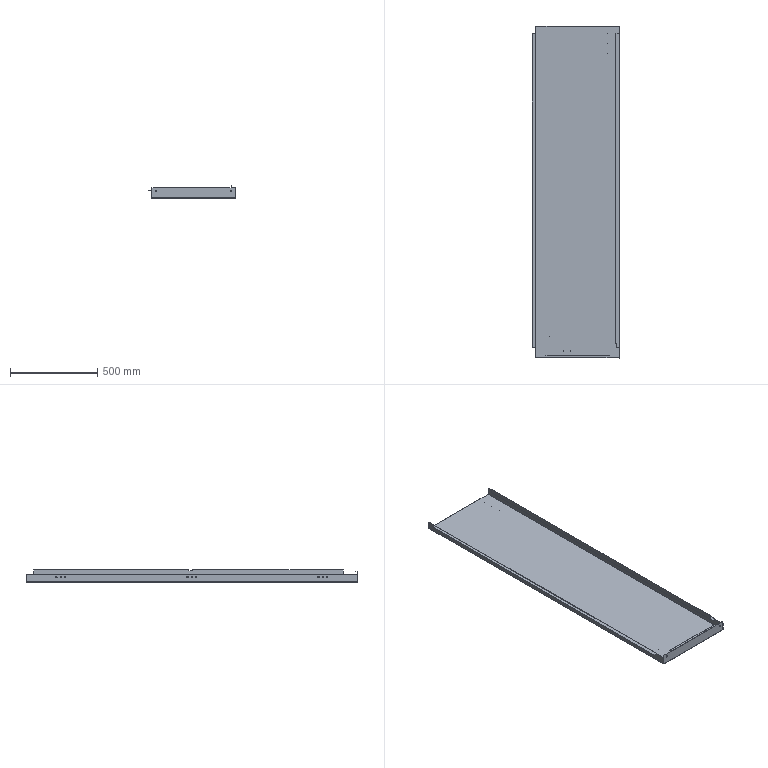Component | SolidWorks | CabinetWelding-1_LeftSidePanel-1 | 1 solid | 130 faces | volume 1463196 mm3 | cylinder 70 | plane 50 | spline 10 | commonest cylinder face diameters 3 x22 7 x18 0.5 x12 0.4 x7 2.8 x7 8.5 x4